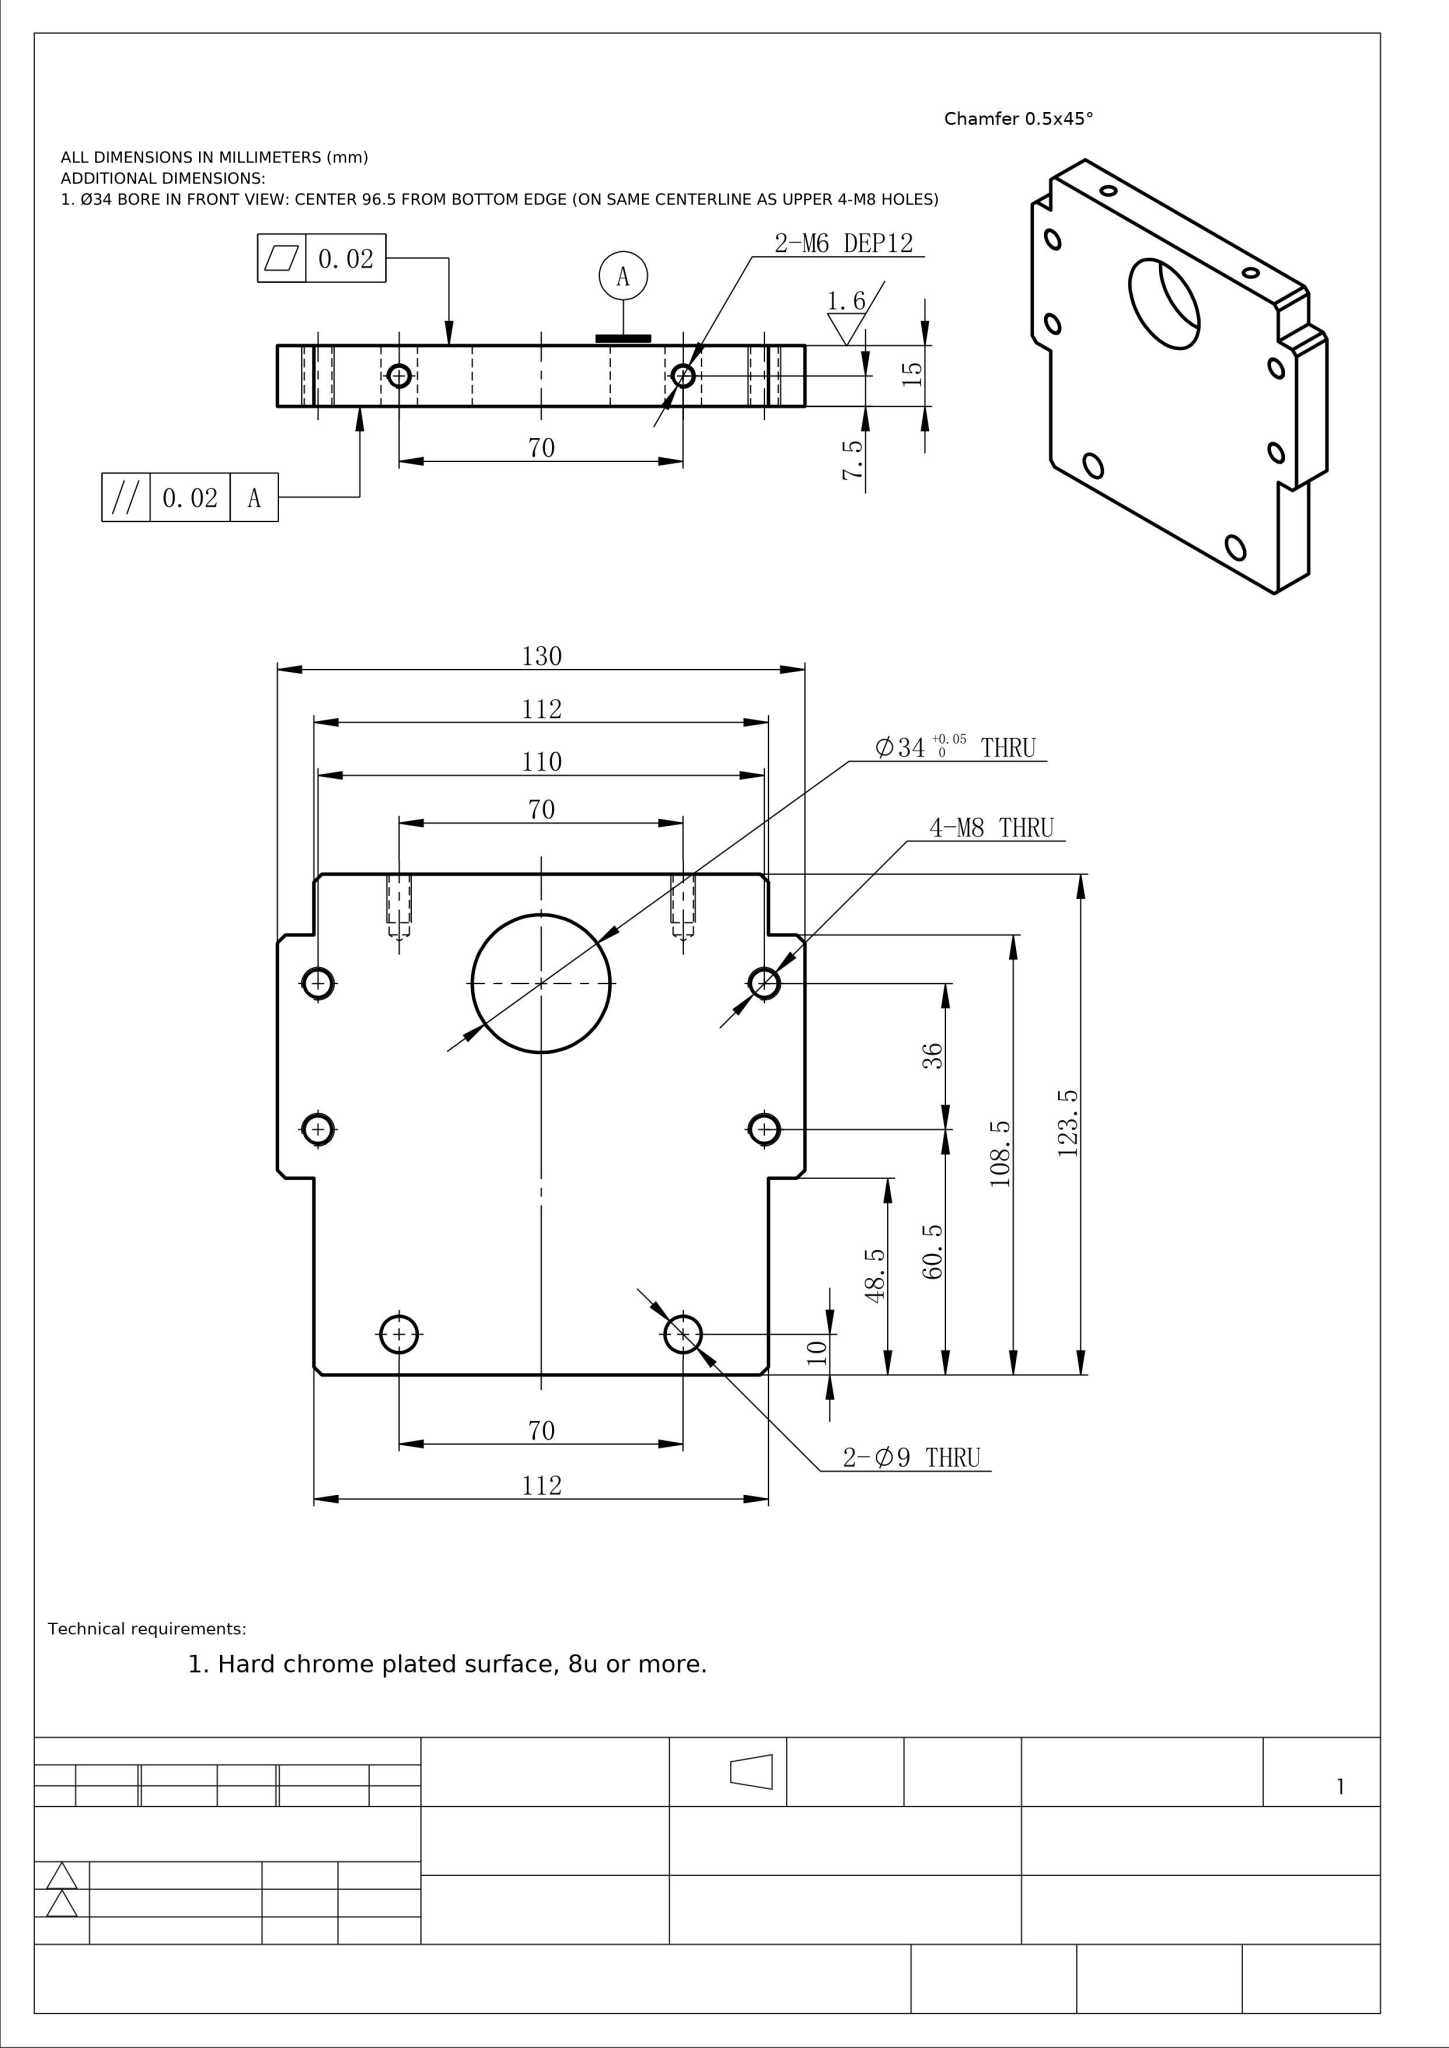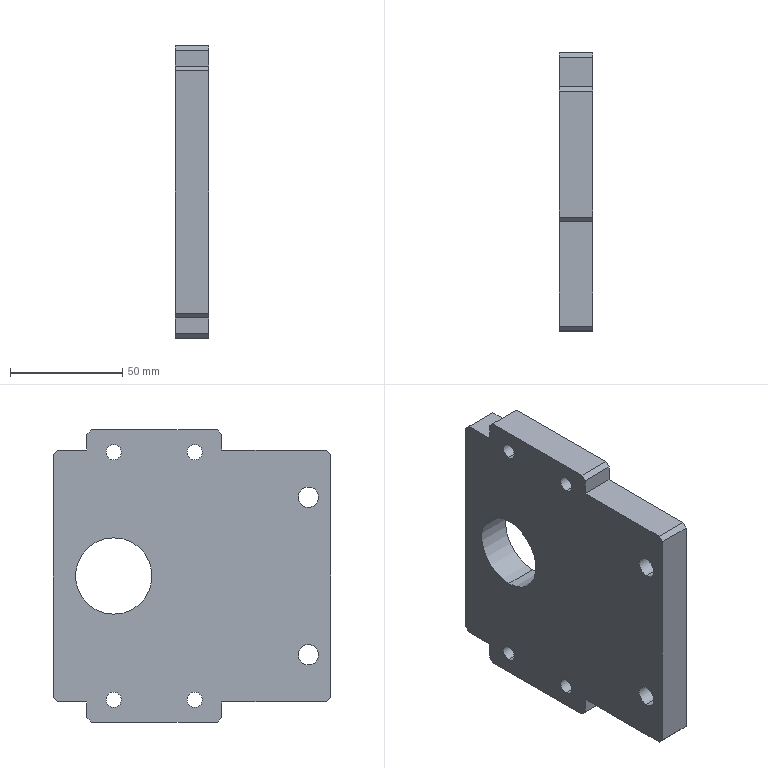Part | NX | mm | 1 solid | 44 faces | box 15 x 123.5 x 130 mm | volume 205125 mm3 | plane 22 | cylinder 18 | cone 4 | commonest cylinder face diameters 6.8 x8 5 x4 9 x4 34 x2